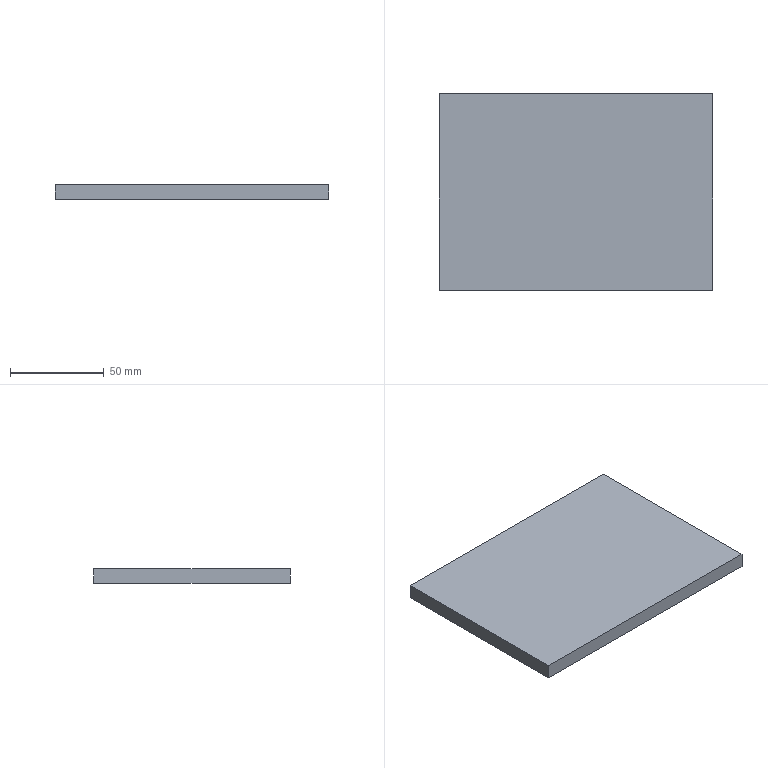Component | SolidWorks | THK-A1024DrivenWheelBracketFrontPlate-1 | 1 solid | 6 faces | box 146 x 105 x 8 mm | volume 122640 mm3 | plane 6 | material Q235A
build123d program:
from build123d import *

# Parameters (mm, degrees)
SKETCH1_W           = 146
SKETCH1_H           = 105
BOSS_EXTRUDE1_DEPTH = 4


with BuildPart() as part:
    # Sketch1 → Boss-Extrude1 (new, symmetric)
    with BuildSketch(Plane.XY):
        Rectangle(SKETCH1_W, SKETCH1_H)
    extrude(amount=BOSS_EXTRUDE1_DEPTH, both=True)


solid = part.part

# Placed as in the assembly
solid = solid.moved(Location((0, -82.5, -1403), (0, 0, 0)))
STEP:
#1=COLOUR_RGB('',0.7922,0.8196,0.9333);
#2=FILL_AREA_STYLE_COLOUR('',#1);
#3=FILL_AREA_STYLE('',(#2));
#4=SURFACE_STYLE_FILL_AREA(#3);
#5=SURFACE_SIDE_STYLE('',(#4));
#6=SURFACE_STYLE_USAGE(.BOTH.,#5);
#7=PRESENTATION_STYLE_ASSIGNMENT((#6));
#8=CARTESIAN_POINT('',(2.874,-5.315,-55.394));
#9=VERTEX_POINT('',#8);
#10=CARTESIAN_POINT('',(2.874,-1.181,-55.394));
#11=VERTEX_POINT('',#10);
#12=CARTESIAN_POINT('',(2.874,-5.315,-55.394));
#13=DIRECTION('',(0.,1.,0.));
#14=VECTOR('',#13,39.37);
#15=LINE('',#12,#14);
#16=EDGE_CURVE('',#9,#11,#15,.T.);
#17=ORIENTED_EDGE('',*,*,#16,.T.);
#18=CARTESIAN_POINT('',(2.874,-1.181,-55.079));
#19=VERTEX_POINT('',#18);
#20=CARTESIAN_POINT('',(2.874,-1.181,-55.079));
#21=DIRECTION('',(0.,0.,-1.));
#22=VECTOR('',#21,39.37);
#23=LINE('',#20,#22);
#24=EDGE_CURVE('',#19,#11,#23,.T.);
#25=ORIENTED_EDGE('',*,*,#24,.F.);
#26=CARTESIAN_POINT('',(2.874,-5.315,-55.079));
#27=VERTEX_POINT('',#26);
#28=CARTESIAN_POINT('',(2.874,-5.315,-55.079));
#29=DIRECTION('',(0.,1.,0.));
#30=VECTOR('',#29,39.37);
#31=LINE('',#28,#30);
#32=EDGE_CURVE('',#27,#19,#31,.T.);
#33=ORIENTED_EDGE('',*,*,#32,.F.);
#34=CARTESIAN_POINT('',(2.874,-5.315,-55.079));
#35=DIRECTION('',(0.,0.,-1.));
#36=VECTOR('',#35,39.37);
#37=LINE('',#34,#36);
#38=EDGE_CURVE('',#27,#9,#37,.T.);
#39=ORIENTED_EDGE('',*,*,#38,.T.);
#40=EDGE_LOOP('',(#17,#25,#33,#39));
#41=FACE_OUTER_BOUND('',#40,.T.);
#42=CARTESIAN_POINT('',(2.874,-5.315,-55.079));
#43=DIRECTION('',(-1.,0.,0.));
#44=DIRECTION('',(0.,0.,1.));
#45=AXIS2_PLACEMENT_3D('',#42,#43,#44);
#46=PLANE('',#45);
#47=ADVANCED_FACE('',(#41),#46,.F.);
#48=CARTESIAN_POINT('',(-2.874,-1.181,-55.394));
#49=VERTEX_POINT('',#48);
#50=CARTESIAN_POINT('',(-2.874,-1.181,-55.394));
#51=DIRECTION('',(-1.,0.,0.));
#52=VECTOR('',#51,39.37);
#53=LINE('',#50,#52);
#54=EDGE_CURVE('',#11,#49,#53,.T.);
#55=ORIENTED_EDGE('',*,*,#54,.T.);
#56=CARTESIAN_POINT('',(-2.874,-1.181,-55.079));
#57=VERTEX_POINT('',#56);
#58=CARTESIAN_POINT('',(-2.874,-1.181,-55.079));
#59=DIRECTION('',(0.,0.,-1.));
#60=VECTOR('',#59,39.37);
#61=LINE('',#58,#60);
#62=EDGE_CURVE('',#57,#49,#61,.T.);
#63=ORIENTED_EDGE('',*,*,#62,.F.);
#64=CARTESIAN_POINT('',(-2.874,-1.181,-55.079));
#65=DIRECTION('',(-1.,0.,0.));
#66=VECTOR('',#65,39.37);
#67=LINE('',#64,#66);
#68=EDGE_CURVE('',#19,#57,#67,.T.);
#69=ORIENTED_EDGE('',*,*,#68,.F.);
#70=ORIENTED_EDGE('',*,*,#24,.T.);
#71=EDGE_LOOP('',(#55,#63,#69,#70));
#72=FACE_OUTER_BOUND('',#71,.T.);
#73=CARTESIAN_POINT('',(-2.874,-1.181,-55.079));
#74=DIRECTION('',(0.,-1.,0.));
#75=DIRECTION('',(0.,0.,-1.));
#76=AXIS2_PLACEMENT_3D('',#73,#74,#75);
#77=PLANE('',#76);
#78=ADVANCED_FACE('',(#72),#77,.F.);
#79=CARTESIAN_POINT('',(-2.874,-5.315,-55.394));
#80=VERTEX_POINT('',#79);
#81=CARTESIAN_POINT('',(-2.874,-5.315,-55.394));
#82=DIRECTION('',(0.,-1.,0.));
#83=VECTOR('',#82,39.37);
#84=LINE('',#81,#83);
#85=EDGE_CURVE('',#49,#80,#84,.T.);
#86=ORIENTED_EDGE('',*,*,#85,.T.);
#87=CARTESIAN_POINT('',(-2.874,-5.315,-55.079));
#88=VERTEX_POINT('',#87);
#89=CARTESIAN_POINT('',(-2.874,-5.315,-55.079));
#90=DIRECTION('',(0.,0.,-1.));
#91=VECTOR('',#90,39.37);
#92=LINE('',#89,#91);
#93=EDGE_CURVE('',#88,#80,#92,.T.);
#94=ORIENTED_EDGE('',*,*,#93,.F.);
#95=CARTESIAN_POINT('',(-2.874,-5.315,-55.079));
#96=DIRECTION('',(0.,-1.,0.));
#97=VECTOR('',#96,39.37);
#98=LINE('',#95,#97);
#99=EDGE_CURVE('',#57,#88,#98,.T.);
#100=ORIENTED_EDGE('',*,*,#99,.F.);
#101=ORIENTED_EDGE('',*,*,#62,.T.);
#102=EDGE_LOOP('',(#86,#94,#100,#101));
#103=FACE_OUTER_BOUND('',#102,.T.);
#104=CARTESIAN_POINT('',(-2.874,-5.315,-55.079));
#105=DIRECTION('',(1.,0.,0.));
#106=DIRECTION('',(0.,0.,-1.));
#107=AXIS2_PLACEMENT_3D('',#104,#105,#106);
#108=PLANE('',#107);
#109=ADVANCED_FACE('',(#103),#108,.F.);
#110=CARTESIAN_POINT('',(-2.874,-5.315,-55.394));
#111=DIRECTION('',(1.,0.,0.));
#112=VECTOR('',#111,39.37);
#113=LINE('',#110,#112);
#114=EDGE_CURVE('',#80,#9,#113,.T.);
#115=ORIENTED_EDGE('',*,*,#114,.T.);
#116=ORIENTED_EDGE('',*,*,#38,.F.);
#117=CARTESIAN_POINT('',(-2.874,-5.315,-55.079));
#118=DIRECTION('',(1.,0.,0.));
#119=VECTOR('',#118,39.37);
#120=LINE('',#117,#119);
#121=EDGE_CURVE('',#88,#27,#120,.T.);
#122=ORIENTED_EDGE('',*,*,#121,.F.);
#123=ORIENTED_EDGE('',*,*,#93,.T.);
#124=EDGE_LOOP('',(#115,#116,#122,#123));
#125=FACE_OUTER_BOUND('',#124,.T.);
#126=CARTESIAN_POINT('',(-2.874,-5.315,-55.079));
#127=DIRECTION('',(0.,1.,0.));
#128=DIRECTION('',(0.,0.,1.));
#129=AXIS2_PLACEMENT_3D('',#126,#127,#128);
#130=PLANE('',#129);
#131=ADVANCED_FACE('',(#125),#130,.F.);
#132=ORIENTED_EDGE('',*,*,#32,.T.);
#133=ORIENTED_EDGE('',*,*,#68,.T.);
#134=ORIENTED_EDGE('',*,*,#99,.T.);
#135=ORIENTED_EDGE('',*,*,#121,.T.);
#136=EDGE_LOOP('',(#132,#133,#134,#135));
#137=FACE_OUTER_BOUND('',#136,.T.);
#138=CARTESIAN_POINT('',(-0.,-3.248,-55.079));
#139=DIRECTION('',(0.,0.,-1.));
#140=DIRECTION('',(-1.,0.,0.));
#141=AXIS2_PLACEMENT_3D('',#138,#139,#140);
#142=PLANE('',#141);
#143=ADVANCED_FACE('',(#137),#142,.F.);
#144=ORIENTED_EDGE('',*,*,#16,.F.);
#145=ORIENTED_EDGE('',*,*,#114,.F.);
#146=ORIENTED_EDGE('',*,*,#85,.F.);
#147=ORIENTED_EDGE('',*,*,#54,.F.);
#148=EDGE_LOOP('',(#144,#145,#146,#147));
#149=FACE_OUTER_BOUND('',#148,.T.);
#150=CARTESIAN_POINT('',(-0.,-3.248,-55.394));
#151=DIRECTION('',(0.,0.,-1.));
#152=DIRECTION('',(-1.,0.,0.));
#153=AXIS2_PLACEMENT_3D('',#150,#151,#152);
#154=PLANE('',#153);
#155=ADVANCED_FACE('',(#149),#154,.T.);
#156=CLOSED_SHELL('',(#47,#78,#109,#131,#143,#155));
#157=MANIFOLD_SOLID_BREP('',#156);
#158=STYLED_ITEM('',(#7),#157);
#159=PRESENTATION_LAYER_ASSIGNMENT('','',(#158));
#160=(LENGTH_UNIT()NAMED_UNIT(*)SI_UNIT($,.METRE.));
#161=LENGTH_MEASURE_WITH_UNIT(LENGTH_MEASURE(0.0254),#160);
#162=DIMENSIONAL_EXPONENTS(1.,0.,0.,0.,0.,0.,0.);
#163=(CONVERSION_BASED_UNIT('',#161)LENGTH_UNIT()NAMED_UNIT(#162));
#164=UNCERTAINTY_MEASURE_WITH_UNIT(LENGTH_MEASURE(0.00001),#163,'','');
#165=(NAMED_UNIT(*)PLANE_ANGLE_UNIT()SI_UNIT($,.RADIAN.));
#166=(NAMED_UNIT(*)SI_UNIT($,.STERADIAN.)SOLID_ANGLE_UNIT());
#167=(GEOMETRIC_REPRESENTATION_CONTEXT(3)GLOBAL_UNCERTAINTY_ASSIGNED_CONTEXT((#164))GLOBAL_UNIT_ASSIGNED_CONTEXT((#163,#165,#166))REPRESENTATION_CONTEXT('',''));
#168=MECHANICAL_DESIGN_GEOMETRIC_PRESENTATION_REPRESENTATION('',(#158),#167);
#169=CARTESIAN_POINT('',(0.,0.,0.));
#170=DIRECTION('',(0.,0.,1.));
#171=DIRECTION('',(1.,0.,0.));
#172=AXIS2_PLACEMENT_3D('',#169,#170,#171);
#173=(LENGTH_UNIT()NAMED_UNIT(*)SI_UNIT($,.METRE.));
#174=LENGTH_MEASURE_WITH_UNIT(LENGTH_MEASURE(0.0254),#173);
#175=DIMENSIONAL_EXPONENTS(1.,0.,0.,0.,0.,0.,0.);
#176=(CONVERSION_BASED_UNIT('',#174)LENGTH_UNIT()NAMED_UNIT(#175));
#177=UNCERTAINTY_MEASURE_WITH_UNIT(LENGTH_MEASURE(0.00001),#176,'','');
#178=(NAMED_UNIT(*)PLANE_ANGLE_UNIT()SI_UNIT($,.RADIAN.));
#179=(NAMED_UNIT(*)SI_UNIT($,.STERADIAN.)SOLID_ANGLE_UNIT());
#180=(GEOMETRIC_REPRESENTATION_CONTEXT(3)GLOBAL_UNCERTAINTY_ASSIGNED_CONTEXT((#177))GLOBAL_UNIT_ASSIGNED_CONTEXT((#176,#178,#179))REPRESENTATION_CONTEXT('',''));
#181=ADVANCED_BREP_SHAPE_REPRESENTATION('',(#157,#172),#180);